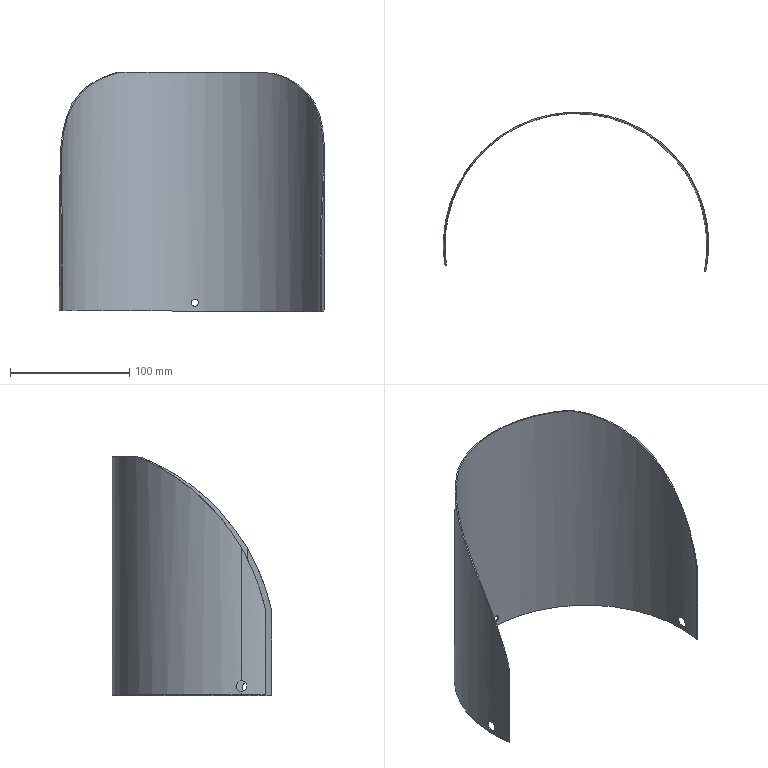Component | SolidWorks | Light-1_Lampshade-2 | 1 solid | 18 faces | volume 67787 mm3 | cylinder 14 | plane 4 | commonest cylinder face diameters 9 x4 220 x3 222 x3 6 x2 359.25 x2